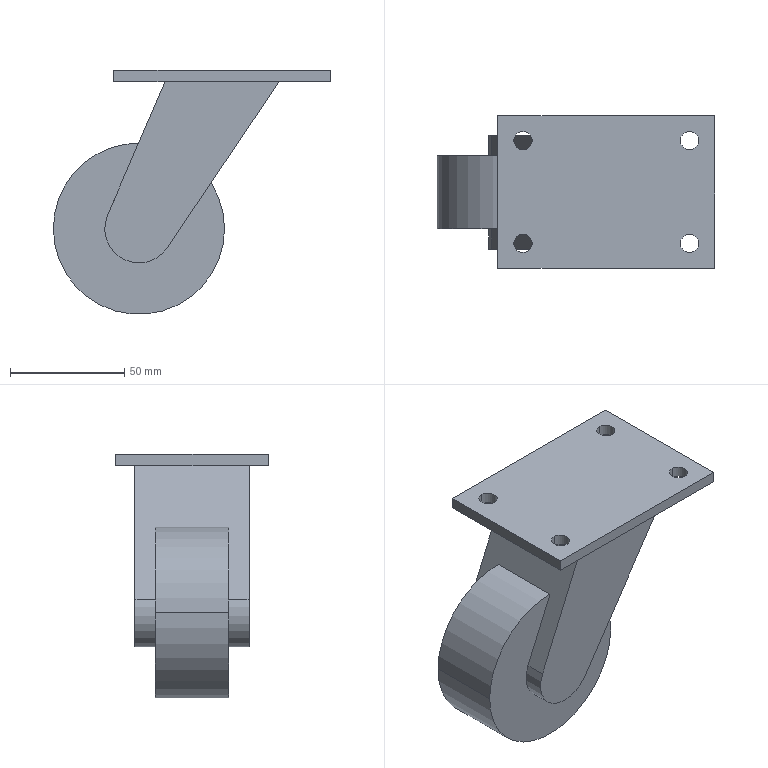Component | SolidWorks | Caster-3 | 1 solid | 25 faces | box 121.5 x 67 x 107 mm | volume 276484 mm3 | cylinder 13 | plane 12 | commonest cylinder face diameters 8 x8 75 x3 30 x2
build123d program:
from build123d import *

# Parameters (mm, degrees)
SKETCH1_R          = 37.5
EXTRUDE1_DEPTH     = 16
SKETCH3_W          = 95
SKETCH3_H          = 5
EXTRUDE2_DEPTH     = 33.5
EXTRUDE3_DEPTH     = 25
CUT_EXTRUDE1_REACH = 142.097
SKETCH5_R          = 4


with BuildPart() as part:
    # Sketch1 → Extrude1 (new, symmetric)
    with BuildSketch(Plane.XY):
        Circle(SKETCH1_R)
    extrude(amount=EXTRUDE1_DEPTH, both=True)



with BuildPart() as body_2:
    # Sketch3 → Extrude2 (new, symmetric)
    with BuildSketch(Plane.XY):
        with Locations((-36.5, 67)):
            Rectangle(SKETCH3_W, SKETCH3_H)
    extrude(amount=EXTRUDE2_DEPTH, both=True)


with BuildPart() as part_1:
    add(part.part)

    add(body_2.part)  # Extrude3 merges body 2
    # Sketch4 → Extrude3 (add, symmetric)
    with BuildSketch(Plane.XY):
        with BuildLine():
            Line((-61.5, 64.5), (-11.5, 64.5))
            Line((-11.5, 64.5), (13.772, 5.944))
            ThreePointArc((13.772, 5.944), (7.191, -13.164), (-12.443, -8.376))
            Line((-12.443, -8.376), (-61.5, 64.5))
        make_face()
    extrude(amount=EXTRUDE3_DEPTH, both=True)

    # Sketch5 → Cut-Extrude1 (cut, up to next)
    with BuildSketch(Plane(origin=(0, 69.5, 0), x_dir=(-1, 0, 0), z_dir=(0, 1, 0)), mode=Mode.PRIVATE) as cut_extrude1_sk1:
        with Locations(Location((0, -22.5, 0), (0, 0, 90))):
            Circle(SKETCH5_R)
    cut_extrude1_tool1 = extrude(cut_extrude1_sk1.sketch, amount=-CUT_EXTRUDE1_REACH, mode=Mode.PRIVATE) & part_1.part
    # Sketch5 → Cut-Extrude1 (cut, up to next)
    with BuildSketch(Plane(origin=(0, 69.5, 0), x_dir=(-1, 0, 0), z_dir=(0, 1, 0)), mode=Mode.PRIVATE) as cut_extrude1_sk2:
        with Locations(Location((0, 22.5, 0), (0, 0, 90))):
            Circle(SKETCH5_R)
    cut_extrude1_tool2 = extrude(cut_extrude1_sk2.sketch, amount=-CUT_EXTRUDE1_REACH, mode=Mode.PRIVATE) & part_1.part
    # Sketch5 → Cut-Extrude1 (cut, up to next)
    with BuildSketch(Plane(origin=(0, 69.5, 0), x_dir=(-1, 0, 0), z_dir=(0, 1, 0)), mode=Mode.PRIVATE) as cut_extrude1_sk3:
        with Locations(Location((73, 22.5, 0), (0, 0, 90))):
            Circle(SKETCH5_R)
    cut_extrude1_tool3 = extrude(cut_extrude1_sk3.sketch, amount=-CUT_EXTRUDE1_REACH, mode=Mode.PRIVATE) & part_1.part
    # Sketch5 → Cut-Extrude1 (cut, up to next)
    with BuildSketch(Plane(origin=(0, 69.5, 0), x_dir=(-1, 0, 0), z_dir=(0, 1, 0)), mode=Mode.PRIVATE) as cut_extrude1_sk4:
        with Locations(Location((73, -22.5, 0), (0, 0, 90))):
            Circle(SKETCH5_R)
    cut_extrude1_tool4 = extrude(cut_extrude1_sk4.sketch, amount=-CUT_EXTRUDE1_REACH, mode=Mode.PRIVATE) & part_1.part
    add(cut_extrude1_tool1.solids().sort_by_distance((0, 69.5, -22.5))[0], mode=Mode.SUBTRACT)
    add(cut_extrude1_tool2.solids().sort_by_distance((0, 69.5, 22.5))[0], mode=Mode.SUBTRACT)
    add(cut_extrude1_tool3.solids().sort_by_distance((-73, 69.5, 22.5))[0], mode=Mode.SUBTRACT)
    add(cut_extrude1_tool4.solids().sort_by_distance((-73, 69.5, -22.5))[0], mode=Mode.SUBTRACT)


solid = part_1.part

# Placed as in the assembly
solid = solid.moved(Location((-626.868, -171.075, 1106.75), (-90, 0, 180)))
STEP:
#1=CARTESIAN_POINT('',(-21.806,-7.464,46.112));
#2=VERTEX_POINT('',#1);
#3=CARTESIAN_POINT('',(-21.806,-7.779,46.112));
#4=VERTEX_POINT('',#3);
#5=CARTESIAN_POINT('',(-21.806,-7.621,46.112));
#6=DIRECTION('',(-0.,-0.,-1.));
#7=DIRECTION('',(0.,1.,0.));
#8=AXIS2_PLACEMENT_3D('',#5,#6,#7);
#9=CIRCLE('',#8,0.1575);
#10=EDGE_CURVE('',#2,#4,#9,.T.);
#11=ORIENTED_EDGE('',*,*,#10,.T.);
#12=CARTESIAN_POINT('',(-21.806,-7.779,46.309));
#13=VERTEX_POINT('',#12);
#14=CARTESIAN_POINT('',(-21.806,-7.779,42.096));
#15=DIRECTION('',(0.,0.,1.));
#16=VECTOR('',#15,39.37);
#17=LINE('',#14,#16);
#18=EDGE_CURVE('',#4,#13,#17,.T.);
#19=ORIENTED_EDGE('',*,*,#18,.T.);
#20=CARTESIAN_POINT('',(-21.806,-7.464,46.309));
#21=VERTEX_POINT('',#20);
#22=CARTESIAN_POINT('',(-21.806,-7.621,46.309));
#23=DIRECTION('',(0.,0.,1.));
#24=DIRECTION('',(0.,1.,0.));
#25=AXIS2_PLACEMENT_3D('',#22,#23,#24);
#26=CIRCLE('',#25,0.1575);
#27=EDGE_CURVE('',#13,#21,#26,.T.);
#28=ORIENTED_EDGE('',*,*,#27,.T.);
#29=CARTESIAN_POINT('',(-21.806,-7.464,42.096));
#30=DIRECTION('',(0.,0.,1.));
#31=VECTOR('',#30,39.37);
#32=LINE('',#29,#31);
#33=EDGE_CURVE('',#2,#21,#32,.T.);
#34=ORIENTED_EDGE('',*,*,#33,.F.);
#35=EDGE_LOOP('',(#11,#19,#28,#34));
#36=FACE_OUTER_BOUND('',#35,.T.);
#37=CARTESIAN_POINT('',(-21.806,-7.621,42.096));
#38=DIRECTION('',(0.,0.,1.));
#39=DIRECTION('',(0.,1.,0.));
#40=AXIS2_PLACEMENT_3D('',#37,#38,#39);
#41=CYLINDRICAL_SURFACE('',#40,0.1575);
#42=ADVANCED_FACE('',(#36),#41,.F.);
#43=CARTESIAN_POINT('',(-21.806,-5.692,46.112));
#44=VERTEX_POINT('',#43);
#45=CARTESIAN_POINT('',(-21.806,-6.007,46.112));
#46=VERTEX_POINT('',#45);
#47=CARTESIAN_POINT('',(-21.806,-5.849,46.112));
#48=DIRECTION('',(-0.,-0.,-1.));
#49=DIRECTION('',(0.,1.,0.));
#50=AXIS2_PLACEMENT_3D('',#47,#48,#49);
#51=CIRCLE('',#50,0.1575);
#52=EDGE_CURVE('',#44,#46,#51,.T.);
#53=ORIENTED_EDGE('',*,*,#52,.T.);
#54=CARTESIAN_POINT('',(-21.806,-6.007,46.309));
#55=VERTEX_POINT('',#54);
#56=CARTESIAN_POINT('',(-21.806,-6.007,42.096));
#57=DIRECTION('',(0.,0.,1.));
#58=VECTOR('',#57,39.37);
#59=LINE('',#56,#58);
#60=EDGE_CURVE('',#46,#55,#59,.T.);
#61=ORIENTED_EDGE('',*,*,#60,.T.);
#62=CARTESIAN_POINT('',(-21.806,-5.692,46.309));
#63=VERTEX_POINT('',#62);
#64=CARTESIAN_POINT('',(-21.806,-5.849,46.309));
#65=DIRECTION('',(0.,0.,1.));
#66=DIRECTION('',(0.,1.,0.));
#67=AXIS2_PLACEMENT_3D('',#64,#65,#66);
#68=CIRCLE('',#67,0.1575);
#69=EDGE_CURVE('',#55,#63,#68,.T.);
#70=ORIENTED_EDGE('',*,*,#69,.T.);
#71=CARTESIAN_POINT('',(-21.806,-5.692,42.096));
#72=DIRECTION('',(0.,0.,1.));
#73=VECTOR('',#72,39.37);
#74=LINE('',#71,#73);
#75=EDGE_CURVE('',#44,#63,#74,.T.);
#76=ORIENTED_EDGE('',*,*,#75,.F.);
#77=EDGE_LOOP('',(#53,#61,#70,#76));
#78=FACE_OUTER_BOUND('',#77,.T.);
#79=CARTESIAN_POINT('',(-21.806,-5.849,42.096));
#80=DIRECTION('',(0.,0.,1.));
#81=DIRECTION('',(0.,1.,0.));
#82=AXIS2_PLACEMENT_3D('',#79,#80,#81);
#83=CYLINDRICAL_SURFACE('',#82,0.1575);
#84=ADVANCED_FACE('',(#78),#83,.F.);
#85=CARTESIAN_POINT('',(-24.68,-5.692,46.112));
#86=VERTEX_POINT('',#85);
#87=CARTESIAN_POINT('',(-24.68,-6.007,46.112));
#88=VERTEX_POINT('',#87);
#89=CARTESIAN_POINT('',(-24.68,-5.849,46.112));
#90=DIRECTION('',(-0.,-0.,-1.));
#91=DIRECTION('',(0.,1.,0.));
#92=AXIS2_PLACEMENT_3D('',#89,#90,#91);
#93=CIRCLE('',#92,0.1575);
#94=EDGE_CURVE('',#86,#88,#93,.T.);
#95=ORIENTED_EDGE('',*,*,#94,.T.);
#96=CARTESIAN_POINT('',(-24.68,-6.007,46.309));
#97=VERTEX_POINT('',#96);
#98=CARTESIAN_POINT('',(-24.68,-6.007,42.096));
#99=DIRECTION('',(0.,0.,1.));
#100=VECTOR('',#99,39.37);
#101=LINE('',#98,#100);
#102=EDGE_CURVE('',#88,#97,#101,.T.);
#103=ORIENTED_EDGE('',*,*,#102,.T.);
#104=CARTESIAN_POINT('',(-24.68,-5.692,46.309));
#105=VERTEX_POINT('',#104);
#106=CARTESIAN_POINT('',(-24.68,-5.849,46.309));
#107=DIRECTION('',(0.,0.,1.));
#108=DIRECTION('',(0.,1.,0.));
#109=AXIS2_PLACEMENT_3D('',#106,#107,#108);
#110=CIRCLE('',#109,0.1575);
#111=EDGE_CURVE('',#97,#105,#110,.T.);
#112=ORIENTED_EDGE('',*,*,#111,.T.);
#113=CARTESIAN_POINT('',(-24.68,-5.692,42.096));
#114=DIRECTION('',(0.,0.,1.));
#115=VECTOR('',#114,39.37);
#116=LINE('',#113,#115);
#117=EDGE_CURVE('',#86,#105,#116,.T.);
#118=ORIENTED_EDGE('',*,*,#117,.F.);
#119=EDGE_LOOP('',(#95,#103,#112,#118));
#120=FACE_OUTER_BOUND('',#119,.T.);
#121=CARTESIAN_POINT('',(-24.68,-5.849,42.096));
#122=DIRECTION('',(0.,0.,1.));
#123=DIRECTION('',(0.,1.,0.));
#124=AXIS2_PLACEMENT_3D('',#121,#122,#123);
#125=CYLINDRICAL_SURFACE('',#124,0.1575);
#126=ADVANCED_FACE('',(#120),#125,.F.);
#127=CARTESIAN_POINT('',(-24.68,-7.464,46.112));
#128=VERTEX_POINT('',#127);
#129=CARTESIAN_POINT('',(-24.68,-7.779,46.112));
#130=VERTEX_POINT('',#129);
#131=CARTESIAN_POINT('',(-24.68,-7.621,46.112));
#132=DIRECTION('',(-0.,-0.,-1.));
#133=DIRECTION('',(0.,1.,0.));
#134=AXIS2_PLACEMENT_3D('',#131,#132,#133);
#135=CIRCLE('',#134,0.1575);
#136=EDGE_CURVE('',#128,#130,#135,.T.);
#137=ORIENTED_EDGE('',*,*,#136,.T.);
#138=CARTESIAN_POINT('',(-24.68,-7.779,46.309));
#139=VERTEX_POINT('',#138);
#140=CARTESIAN_POINT('',(-24.68,-7.779,42.096));
#141=DIRECTION('',(0.,0.,1.));
#142=VECTOR('',#141,39.37);
#143=LINE('',#140,#142);
#144=EDGE_CURVE('',#130,#139,#143,.T.);
#145=ORIENTED_EDGE('',*,*,#144,.T.);
#146=CARTESIAN_POINT('',(-24.68,-7.464,46.309));
#147=VERTEX_POINT('',#146);
#148=CARTESIAN_POINT('',(-24.68,-7.621,46.309));
#149=DIRECTION('',(0.,0.,1.));
#150=DIRECTION('',(0.,1.,0.));
#151=AXIS2_PLACEMENT_3D('',#148,#149,#150);
#152=CIRCLE('',#151,0.1575);
#153=EDGE_CURVE('',#139,#147,#152,.T.);
#154=ORIENTED_EDGE('',*,*,#153,.T.);
#155=CARTESIAN_POINT('',(-24.68,-7.464,42.096));
#156=DIRECTION('',(0.,0.,1.));
#157=VECTOR('',#156,39.37);
#158=LINE('',#155,#157);
#159=EDGE_CURVE('',#128,#147,#158,.T.);
#160=ORIENTED_EDGE('',*,*,#159,.F.);
#161=EDGE_LOOP('',(#137,#145,#154,#160));
#162=FACE_OUTER_BOUND('',#161,.T.);
#163=CARTESIAN_POINT('',(-24.68,-7.621,42.096));
#164=DIRECTION('',(0.,0.,1.));
#165=DIRECTION('',(0.,1.,0.));
#166=AXIS2_PLACEMENT_3D('',#163,#164,#165);
#167=CYLINDRICAL_SURFACE('',#166,0.1575);
#168=ADVANCED_FACE('',(#162),#167,.F.);
#169=CARTESIAN_POINT('',(-26.156,-6.105,43.573));
#170=VERTEX_POINT('',#169);
#171=CARTESIAN_POINT('',(-24.686,-6.105,45.049));
#172=VERTEX_POINT('',#171);
#173=CARTESIAN_POINT('',(-24.68,-6.105,43.573));
#174=DIRECTION('',(0.,1.,-0.));
#175=DIRECTION('',(-1.,0.,0.));
#176=AXIS2_PLACEMENT_3D('',#173,#174,#175);
#177=CIRCLE('',#176,1.476);
#178=EDGE_CURVE('',#170,#172,#177,.T.);
#179=ORIENTED_EDGE('',*,*,#178,.F.);
#180=CARTESIAN_POINT('',(-26.156,-7.365,43.573));
#181=VERTEX_POINT('',#180);
#182=CARTESIAN_POINT('',(-26.156,-6.105,43.573));
#183=DIRECTION('',(-0.,-1.,0.));
#184=VECTOR('',#183,39.37);
#185=LINE('',#182,#184);
#186=EDGE_CURVE('',#170,#181,#185,.T.);
#187=ORIENTED_EDGE('',*,*,#186,.T.);
#188=CARTESIAN_POINT('',(-24.686,-7.365,45.049));
#189=VERTEX_POINT('',#188);
#190=CARTESIAN_POINT('',(-24.68,-7.365,43.573));
#191=DIRECTION('',(0.,1.,-0.));
#192=DIRECTION('',(-1.,0.,0.));
#193=AXIS2_PLACEMENT_3D('',#190,#191,#192);
#194=CIRCLE('',#193,1.476);
#195=EDGE_CURVE('',#181,#189,#194,.T.);
#196=ORIENTED_EDGE('',*,*,#195,.T.);
#197=CARTESIAN_POINT('',(-24.686,-6.105,45.049));
#198=DIRECTION('',(0.,1.,-0.));
#199=VECTOR('',#198,39.37);
#200=LINE('',#197,#199);
#201=EDGE_CURVE('',#189,#172,#200,.T.);
#202=ORIENTED_EDGE('',*,*,#201,.T.);
#203=EDGE_LOOP('',(#179,#187,#196,#202));
#204=FACE_OUTER_BOUND('',#203,.T.);
#205=CARTESIAN_POINT('',(-24.68,-6.105,43.573));
#206=DIRECTION('',(-0.,-1.,0.));
#207=DIRECTION('',(1.,-0.,0.));
#208=AXIS2_PLACEMENT_3D('',#205,#206,#207);
#209=CYLINDRICAL_SURFACE('',#208,1.476);
#210=ADVANCED_FACE('',(#204),#209,.T.);
#211=ORIENTED_EDGE('',*,*,#186,.F.);
#212=CARTESIAN_POINT('',(-23.203,-6.105,43.573));
#213=VERTEX_POINT('',#212);
#214=CARTESIAN_POINT('',(-24.68,-6.105,43.573));
#215=DIRECTION('',(0.,1.,-0.));
#216=DIRECTION('',(-1.,0.,0.));
#217=AXIS2_PLACEMENT_3D('',#214,#215,#216);
#218=CIRCLE('',#217,1.476);
#219=EDGE_CURVE('',#213,#170,#218,.T.);
#220=ORIENTED_EDGE('',*,*,#219,.F.);
#221=CARTESIAN_POINT('',(-23.203,-7.365,43.573));
#222=VERTEX_POINT('',#221);
#223=CARTESIAN_POINT('',(-23.203,-6.105,43.573));
#224=DIRECTION('',(-0.,-1.,0.));
#225=VECTOR('',#224,39.37);
#226=LINE('',#223,#225);
#227=EDGE_CURVE('',#213,#222,#226,.T.);
#228=ORIENTED_EDGE('',*,*,#227,.T.);
#229=CARTESIAN_POINT('',(-24.68,-7.365,43.573));
#230=DIRECTION('',(0.,1.,-0.));
#231=DIRECTION('',(-1.,0.,0.));
#232=AXIS2_PLACEMENT_3D('',#229,#230,#231);
#233=CIRCLE('',#232,1.476);
#234=EDGE_CURVE('',#222,#181,#233,.T.);
#235=ORIENTED_EDGE('',*,*,#234,.T.);
#236=EDGE_LOOP('',(#211,#220,#228,#235));
#237=FACE_OUTER_BOUND('',#236,.T.);
#238=CARTESIAN_POINT('',(-24.68,-6.105,43.573));
#239=DIRECTION('',(-0.,-1.,0.));
#240=DIRECTION('',(1.,-0.,0.));
#241=AXIS2_PLACEMENT_3D('',#238,#239,#240);
#242=CYLINDRICAL_SURFACE('',#241,1.476);
#243=ADVANCED_FACE('',(#237),#242,.T.);
#244=CARTESIAN_POINT('',(-24.19,-7.365,43.243));
#245=VERTEX_POINT('',#244);
#246=CARTESIAN_POINT('',(-25.222,-7.365,43.807));
#247=VERTEX_POINT('',#246);
#248=CARTESIAN_POINT('',(-24.68,-7.365,43.573));
#249=DIRECTION('',(0.,1.,-0.));
#250=DIRECTION('',(-1.,0.,0.));
#251=AXIS2_PLACEMENT_3D('',#248,#249,#250);
#252=CIRCLE('',#251,0.5906);
#253=EDGE_CURVE('',#245,#247,#252,.T.);
#254=ORIENTED_EDGE('',*,*,#253,.F.);
#255=CARTESIAN_POINT('',(-24.19,-7.72,43.243));
#256=VERTEX_POINT('',#255);
#257=CARTESIAN_POINT('',(-24.19,-5.751,43.243));
#258=DIRECTION('',(-0.,-1.,0.));
#259=VECTOR('',#258,39.37);
#260=LINE('',#257,#259);
#261=EDGE_CURVE('',#245,#256,#260,.T.);
#262=ORIENTED_EDGE('',*,*,#261,.T.);
#263=CARTESIAN_POINT('',(-25.222,-7.72,43.807));
#264=VERTEX_POINT('',#263);
#265=CARTESIAN_POINT('',(-24.68,-7.72,43.573));
#266=DIRECTION('',(0.,1.,-0.));
#267=DIRECTION('',(-1.,0.,0.));
#268=AXIS2_PLACEMENT_3D('',#265,#266,#267);
#269=CIRCLE('',#268,0.5906);
#270=EDGE_CURVE('',#256,#264,#269,.T.);
#271=ORIENTED_EDGE('',*,*,#270,.T.);
#272=CARTESIAN_POINT('',(-25.222,-5.751,43.807));
#273=DIRECTION('',(-0.,-1.,0.));
#274=VECTOR('',#273,39.37);
#275=LINE('',#272,#274);
#276=EDGE_CURVE('',#247,#264,#275,.T.);
#277=ORIENTED_EDGE('',*,*,#276,.F.);
#278=EDGE_LOOP('',(#254,#262,#271,#277));
#279=FACE_OUTER_BOUND('',#278,.T.);
#280=CARTESIAN_POINT('',(-24.68,-5.751,43.573));
#281=DIRECTION('',(-0.,-1.,0.));
#282=DIRECTION('',(1.,-0.,0.));
#283=AXIS2_PLACEMENT_3D('',#280,#281,#282);
#284=CYLINDRICAL_SURFACE('',#283,0.5906);
#285=ADVANCED_FACE('',(#279),#284,.T.);
#286=CARTESIAN_POINT('',(-21.373,-8.054,46.309));
#287=VERTEX_POINT('',#286);
#288=CARTESIAN_POINT('',(-21.373,-8.054,46.112));
#289=VERTEX_POINT('',#288);
#290=CARTESIAN_POINT('',(-21.373,-8.054,46.309));
#291=DIRECTION('',(-0.,-0.,-1.));
#292=VECTOR('',#291,39.37);
#293=LINE('',#290,#292);
#294=EDGE_CURVE('',#287,#289,#293,.T.);
#295=ORIENTED_EDGE('',*,*,#294,.T.);
#296=CARTESIAN_POINT('',(-21.373,-5.416,46.112));
#297=VERTEX_POINT('',#296);
#298=CARTESIAN_POINT('',(-21.373,-5.416,46.112));
#299=DIRECTION('',(-0.,-1.,0.));
#300=VECTOR('',#299,39.37);
#301=LINE('',#298,#300);
#302=EDGE_CURVE('',#297,#289,#301,.T.);
#303=ORIENTED_EDGE('',*,*,#302,.F.);
#304=CARTESIAN_POINT('',(-21.373,-5.416,46.309));
#305=VERTEX_POINT('',#304);
#306=CARTESIAN_POINT('',(-21.373,-5.416,46.309));
#307=DIRECTION('',(-0.,-0.,-1.));
#308=VECTOR('',#307,39.37);
#309=LINE('',#306,#308);
#310=EDGE_CURVE('',#305,#297,#309,.T.);
#311=ORIENTED_EDGE('',*,*,#310,.F.);
#312=CARTESIAN_POINT('',(-21.373,-5.416,46.309));
#313=DIRECTION('',(-0.,-1.,0.));
#314=VECTOR('',#313,39.37);
#315=LINE('',#312,#314);
#316=EDGE_CURVE('',#305,#287,#315,.T.);
#317=ORIENTED_EDGE('',*,*,#316,.T.);
#318=EDGE_LOOP('',(#295,#303,#311,#317));
#319=FACE_OUTER_BOUND('',#318,.T.);
#320=CARTESIAN_POINT('',(-21.373,-5.416,46.309));
#321=DIRECTION('',(-1.,0.,0.));
#322=DIRECTION('',(-0.,-1.,0.));
#323=AXIS2_PLACEMENT_3D('',#320,#321,#322);
#324=PLANE('',#323);
#325=ADVANCED_FACE('',(#319),#324,.F.);
#326=ORIENTED_EDGE('',*,*,#10,.F.);
#327=CARTESIAN_POINT('',(-21.806,-7.621,46.112));
#328=DIRECTION('',(-0.,-0.,-1.));
#329=DIRECTION('',(0.,1.,0.));
#330=AXIS2_PLACEMENT_3D('',#327,#328,#329);
#331=CIRCLE('',#330,0.1575);
#332=EDGE_CURVE('',#4,#2,#331,.T.);
#333=ORIENTED_EDGE('',*,*,#332,.F.);
#334=EDGE_LOOP('',(#326,#333));
#335=FACE_BOUND('',#334,.T.);
#336=ORIENTED_EDGE('',*,*,#52,.F.);
#337=CARTESIAN_POINT('',(-21.806,-5.849,46.112));
#338=DIRECTION('',(-0.,-0.,-1.));
#339=DIRECTION('',(0.,1.,0.));
#340=AXIS2_PLACEMENT_3D('',#337,#338,#339);
#341=CIRCLE('',#340,0.1575);
#342=EDGE_CURVE('',#46,#44,#341,.T.);
#343=ORIENTED_EDGE('',*,*,#342,.F.);
#344=EDGE_LOOP('',(#336,#343));
#345=FACE_BOUND('',#344,.T.);
#346=ORIENTED_EDGE('',*,*,#94,.F.);
#347=CARTESIAN_POINT('',(-24.68,-5.849,46.112));
#348=DIRECTION('',(-0.,-0.,-1.));
#349=DIRECTION('',(0.,1.,0.));
#350=AXIS2_PLACEMENT_3D('',#347,#348,#349);
#351=CIRCLE('',#350,0.1575);
#352=EDGE_CURVE('',#88,#86,#351,.T.);
#353=ORIENTED_EDGE('',*,*,#352,.F.);
#354=EDGE_LOOP('',(#346,#353));
#355=FACE_BOUND('',#354,.T.);
#356=ORIENTED_EDGE('',*,*,#136,.F.);
#357=CARTESIAN_POINT('',(-24.68,-7.621,46.112));
#358=DIRECTION('',(-0.,-0.,-1.));
#359=DIRECTION('',(0.,1.,0.));
#360=AXIS2_PLACEMENT_3D('',#357,#358,#359);
#361=CIRCLE('',#360,0.1575);
#362=EDGE_CURVE('',#130,#128,#361,.T.);
#363=ORIENTED_EDGE('',*,*,#362,.F.);
#364=EDGE_LOOP('',(#356,#363));
#365=FACE_BOUND('',#364,.T.);
#366=CARTESIAN_POINT('',(-22.259,-5.751,46.112));
#367=VERTEX_POINT('',#366);
#368=CARTESIAN_POINT('',(-22.259,-7.72,46.112));
#369=VERTEX_POINT('',#368);
#370=CARTESIAN_POINT('',(-22.259,-5.751,46.112));
#371=DIRECTION('',(-0.,-1.,0.));
#372=VECTOR('',#371,39.37);
#373=LINE('',#370,#372);
#374=EDGE_CURVE('',#367,#369,#373,.T.);
#375=ORIENTED_EDGE('',*,*,#374,.F.);
#376=CARTESIAN_POINT('',(-24.227,-5.751,46.112));
#377=VERTEX_POINT('',#376);
#378=CARTESIAN_POINT('',(-22.259,-5.751,46.112));
#379=DIRECTION('',(1.,-0.,-0.));
#380=VECTOR('',#379,39.37);
#381=LINE('',#378,#380);
#382=EDGE_CURVE('',#377,#367,#381,.T.);
#383=ORIENTED_EDGE('',*,*,#382,.F.);
#384=CARTESIAN_POINT('',(-24.227,-7.72,46.112));
#385=VERTEX_POINT('',#384);
#386=CARTESIAN_POINT('',(-24.227,-5.751,46.112));
#387=DIRECTION('',(-0.,-1.,0.));
#388=VECTOR('',#387,39.37);
#389=LINE('',#386,#388);
#390=EDGE_CURVE('',#377,#385,#389,.T.);
#391=ORIENTED_EDGE('',*,*,#390,.T.);
#392=CARTESIAN_POINT('',(-22.259,-7.72,46.112));
#393=DIRECTION('',(1.,-0.,-0.));
#394=VECTOR('',#393,39.37);
#395=LINE('',#392,#394);
#396=EDGE_CURVE('',#385,#369,#395,.T.);
#397=ORIENTED_EDGE('',*,*,#396,.T.);
#398=EDGE_LOOP('',(#375,#383,#391,#397));
#399=FACE_BOUND('',#398,.T.);
#400=CARTESIAN_POINT('',(-25.113,-8.054,46.112));
#401=VERTEX_POINT('',#400);
#402=CARTESIAN_POINT('',(-21.373,-8.054,46.112));
#403=DIRECTION('',(-1.,0.,0.));
#404=VECTOR('',#403,39.37);
#405=LINE('',#402,#404);
#406=EDGE_CURVE('',#289,#401,#405,.T.);
#407=ORIENTED_EDGE('',*,*,#406,.T.);
#408=CARTESIAN_POINT('',(-25.113,-5.416,46.112));
#409=VERTEX_POINT('',#408);
#410=CARTESIAN_POINT('',(-25.113,-5.416,46.112));
#411=DIRECTION('',(-0.,-1.,0.));
#412=VECTOR('',#411,39.37);
#413=LINE('',#410,#412);
#414=EDGE_CURVE('',#409,#401,#413,.T.);
#415=ORIENTED_EDGE('',*,*,#414,.F.);
#416=CARTESIAN_POINT('',(-21.373,-5.416,46.112));
#417=DIRECTION('',(-1.,0.,0.));
#418=VECTOR('',#417,39.37);
#419=LINE('',#416,#418);
#420=EDGE_CURVE('',#297,#409,#419,.T.);
#421=ORIENTED_EDGE('',*,*,#420,.F.);
#422=ORIENTED_EDGE('',*,*,#302,.T.);
#423=EDGE_LOOP('',(#407,#415,#421,#422));
#424=FACE_OUTER_BOUND('',#423,.T.);
#425=CARTESIAN_POINT('',(-21.373,-5.416,46.112));
#426=DIRECTION('',(0.,0.,1.));
#427=DIRECTION('',(0.,1.,-0.));
#428=AXIS2_PLACEMENT_3D('',#425,#426,#427);
#429=PLANE('',#428);
#430=ADVANCED_FACE('',(#335,#345,#355,#365,#399,#424),#429,.F.);
#431=CARTESIAN_POINT('',(-25.113,-8.054,46.309));
#432=VERTEX_POINT('',#431);
#433=CARTESIAN_POINT('',(-25.113,-8.054,46.309));
#434=DIRECTION('',(0.,0.,1.));
#435=VECTOR('',#434,39.37);
#436=LINE('',#433,#435);
#437=EDGE_CURVE('',#401,#432,#436,.T.);
#438=ORIENTED_EDGE('',*,*,#437,.T.);
#439=CARTESIAN_POINT('',(-25.113,-5.416,46.309));
#440=VERTEX_POINT('',#439);
#441=CARTESIAN_POINT('',(-25.113,-5.416,46.309));
#442=DIRECTION('',(-0.,-1.,0.));
#443=VECTOR('',#442,39.37);
#444=LINE('',#441,#443);
#445=EDGE_CURVE('',#440,#432,#444,.T.);
#446=ORIENTED_EDGE('',*,*,#445,.F.);
#447=CARTESIAN_POINT('',(-25.113,-5.416,46.309));
#448=DIRECTION('',(0.,0.,1.));
#449=VECTOR('',#448,39.37);
#450=LINE('',#447,#449);
#451=EDGE_CURVE('',#409,#440,#450,.T.);
#452=ORIENTED_EDGE('',*,*,#451,.F.);
#453=ORIENTED_EDGE('',*,*,#414,.T.);
#454=EDGE_LOOP('',(#438,#446,#452,#453));
#455=FACE_OUTER_BOUND('',#454,.T.);
#456=CARTESIAN_POINT('',(-25.113,-5.416,46.309));
#457=DIRECTION('',(1.,-0.,-0.));
#458=DIRECTION('',(0.,1.,-0.));
#459=AXIS2_PLACEMENT_3D('',#456,#457,#458);
#460=PLANE('',#459);
#461=ADVANCED_FACE('',(#455),#460,.F.);
#462=CARTESIAN_POINT('',(-21.806,-7.621,46.309));
#463=DIRECTION('',(0.,0.,1.));
#464=DIRECTION('',(0.,1.,0.));
#465=AXIS2_PLACEMENT_3D('',#462,#463,#464);
#466=CIRCLE('',#465,0.1575);
#467=EDGE_CURVE('',#21,#13,#466,.T.);
#468=ORIENTED_EDGE('',*,*,#467,.F.);
#469=ORIENTED_EDGE('',*,*,#27,.F.);
#470=EDGE_LOOP('',(#468,#469));
#471=FACE_BOUND('',#470,.T.);
#472=CARTESIAN_POINT('',(-21.806,-5.849,46.309));
#473=DIRECTION('',(0.,0.,1.));
#474=DIRECTION('',(0.,1.,0.));
#475=AXIS2_PLACEMENT_3D('',#472,#473,#474);
#476=CIRCLE('',#475,0.1575);
#477=EDGE_CURVE('',#63,#55,#476,.T.);
#478=ORIENTED_EDGE('',*,*,#477,.F.);
#479=ORIENTED_EDGE('',*,*,#69,.F.);
#480=EDGE_LOOP('',(#478,#479));
#481=FACE_BOUND('',#480,.T.);
#482=CARTESIAN_POINT('',(-24.68,-5.849,46.309));
#483=DIRECTION('',(0.,0.,1.));
#484=DIRECTION('',(0.,1.,0.));
#485=AXIS2_PLACEMENT_3D('',#482,#483,#484);
#486=CIRCLE('',#485,0.1575);
#487=EDGE_CURVE('',#105,#97,#486,.T.);
#488=ORIENTED_EDGE('',*,*,#487,.F.);
#489=ORIENTED_EDGE('',*,*,#111,.F.);
#490=EDGE_LOOP('',(#488,#489));
#491=FACE_BOUND('',#490,.T.);
#492=CARTESIAN_POINT('',(-24.68,-7.621,46.309));
#493=DIRECTION('',(0.,0.,1.));
#494=DIRECTION('',(0.,1.,0.));
#495=AXIS2_PLACEMENT_3D('',#492,#493,#494);
#496=CIRCLE('',#495,0.1575);
#497=EDGE_CURVE('',#147,#139,#496,.T.);
#498=ORIENTED_EDGE('',*,*,#497,.F.);
#499=ORIENTED_EDGE('',*,*,#153,.F.);
#500=EDGE_LOOP('',(#498,#499));
#501=FACE_BOUND('',#500,.T.);
#502=CARTESIAN_POINT('',(-21.373,-8.054,46.309));
#503=DIRECTION('',(1.,-0.,-0.));
#504=VECTOR('',#503,39.37);
#505=LINE('',#502,#504);
#506=EDGE_CURVE('',#432,#287,#505,.T.);
#507=ORIENTED_EDGE('',*,*,#506,.T.);
#508=ORIENTED_EDGE('',*,*,#316,.F.);
#509=CARTESIAN_POINT('',(-21.373,-5.416,46.309));
#510=DIRECTION('',(1.,-0.,-0.));
#511=VECTOR('',#510,39.37);
#512=LINE('',#509,#511);
#513=EDGE_CURVE('',#440,#305,#512,.T.);
#514=ORIENTED_EDGE('',*,*,#513,.F.);
#515=ORIENTED_EDGE('',*,*,#445,.T.);
#516=EDGE_LOOP('',(#507,#508,#514,#515));
#517=FACE_OUTER_BOUND('',#516,.T.);
#518=CARTESIAN_POINT('',(-21.373,-5.416,46.309));
#519=DIRECTION('',(-0.,-0.,-1.));
#520=DIRECTION('',(-0.,-1.,0.));
#521=AXIS2_PLACEMENT_3D('',#518,#519,#520);
#522=PLANE('',#521);
#523=ADVANCED_FACE('',(#471,#481,#491,#501,#517),#522,.F.);
#524=ORIENTED_EDGE('',*,*,#310,.T.);
#525=ORIENTED_EDGE('',*,*,#420,.T.);
#526=ORIENTED_EDGE('',*,*,#451,.T.);
#527=ORIENTED_EDGE('',*,*,#513,.T.);
#528=EDGE_LOOP('',(#524,#525,#526,#527));
#529=FACE_OUTER_BOUND('',#528,.T.);
#530=CARTESIAN_POINT('',(-21.373,-5.416,46.112));
#531=DIRECTION('',(0.,1.,-0.));
#532=DIRECTION('',(-1.,0.,0.));
#533=AXIS2_PLACEMENT_3D('',#530,#531,#532);
#534=PLANE('',#533);
#535=ADVANCED_FACE('',(#529),#534,.T.);
#536=ORIENTED_EDGE('',*,*,#294,.F.);
#537=ORIENTED_EDGE('',*,*,#506,.F.);
#538=ORIENTED_EDGE('',*,*,#437,.F.);
#539=ORIENTED_EDGE('',*,*,#406,.F.);
#540=EDGE_LOOP('',(#536,#537,#538,#539));
#541=FACE_OUTER_BOUND('',#540,.T.);
#542=CARTESIAN_POINT('',(-21.373,-8.054,46.112));
#543=DIRECTION('',(0.,1.,-0.));
#544=DIRECTION('',(-1.,0.,0.));
#545=AXIS2_PLACEMENT_3D('',#542,#543,#544);
#546=PLANE('',#545);
#547=ADVANCED_FACE('',(#541),#546,.F.);
#548=CARTESIAN_POINT('',(-23.434,-6.105,44.366));
#549=VERTEX_POINT('',#548);
#550=CARTESIAN_POINT('',(-23.434,-7.365,44.366));
#551=VERTEX_POINT('',#550);
#552=CARTESIAN_POINT('',(-23.434,-6.105,44.366));
#553=DIRECTION('',(-0.,-1.,0.));
#554=VECTOR('',#553,39.37);
#555=LINE('',#552,#554);
#556=EDGE_CURVE('',#549,#551,#555,.T.);
#557=ORIENTED_EDGE('',*,*,#556,.F.);
#558=CARTESIAN_POINT('',(-24.19,-6.105,43.243));
#559=VERTEX_POINT('',#558);
#560=CARTESIAN_POINT('',(-22.259,-6.105,46.112));
#561=DIRECTION('',(-0.5584,0.,-0.8296));
#562=VECTOR('',#561,39.37);
#563=LINE('',#560,#562);
#564=EDGE_CURVE('',#549,#559,#563,.T.);
#565=ORIENTED_EDGE('',*,*,#564,.T.);
#566=CARTESIAN_POINT('',(-24.19,-5.751,43.243));
#567=VERTEX_POINT('',#566);
#568=CARTESIAN_POINT('',(-24.19,-5.751,43.243));
#569=DIRECTION('',(-0.,-1.,0.));
#570=VECTOR('',#569,39.37);
#571=LINE('',#568,#570);
#572=EDGE_CURVE('',#567,#559,#571,.T.);
#573=ORIENTED_EDGE('',*,*,#572,.F.);
#574=CARTESIAN_POINT('',(-22.259,-5.751,46.112));
#575=DIRECTION('',(-0.5584,0.,-0.8296));
#576=VECTOR('',#575,39.37);
#577=LINE('',#574,#576);
#578=EDGE_CURVE('',#367,#567,#577,.T.);
#579=ORIENTED_EDGE('',*,*,#578,.F.);
#580=ORIENTED_EDGE('',*,*,#374,.T.);
#581=CARTESIAN_POINT('',(-22.259,-7.72,46.112));
#582=DIRECTION('',(-0.5584,0.,-0.8296));
#583=VECTOR('',#582,39.37);
#584=LINE('',#581,#583);
#585=EDGE_CURVE('',#369,#256,#584,.T.);
#586=ORIENTED_EDGE('',*,*,#585,.T.);
#587=ORIENTED_EDGE('',*,*,#261,.F.);
#588=CARTESIAN_POINT('',(-22.259,-7.365,46.112));
#589=DIRECTION('',(-0.5584,0.,-0.8296));
#590=VECTOR('',#589,39.37);
#591=LINE('',#588,#590);
#592=EDGE_CURVE('',#551,#245,#591,.T.);
#593=ORIENTED_EDGE('',*,*,#592,.F.);
#594=EDGE_LOOP('',(#557,#565,#573,#579,#580,#586,#587,#593));
#595=FACE_OUTER_BOUND('',#594,.T.);
#596=CARTESIAN_POINT('',(-22.259,-5.751,46.112));
#597=DIRECTION('',(-0.8296,0.,0.5584));
#598=DIRECTION('',(0.5584,-0.,0.8296));
#599=AXIS2_PLACEMENT_3D('',#596,#597,#598);
#600=PLANE('',#599);
#601=ADVANCED_FACE('',(#595),#600,.F.);
#602=ORIENTED_EDGE('',*,*,#572,.T.);
#603=CARTESIAN_POINT('',(-25.222,-6.105,43.807));
#604=VERTEX_POINT('',#603);
#605=CARTESIAN_POINT('',(-24.68,-6.105,43.573));
#606=DIRECTION('',(0.,1.,-0.));
#607=DIRECTION('',(-1.,0.,0.));
#608=AXIS2_PLACEMENT_3D('',#605,#606,#607);
#609=CIRCLE('',#608,0.5906);
#610=EDGE_CURVE('',#559,#604,#609,.T.);
#611=ORIENTED_EDGE('',*,*,#610,.T.);
#612=CARTESIAN_POINT('',(-25.222,-5.751,43.807));
#613=VERTEX_POINT('',#612);
#614=CARTESIAN_POINT('',(-25.222,-5.751,43.807));
#615=DIRECTION('',(-0.,-1.,0.));
#616=VECTOR('',#615,39.37);
#617=LINE('',#614,#616);
#618=EDGE_CURVE('',#613,#604,#617,.T.);
#619=ORIENTED_EDGE('',*,*,#618,.F.);
#620=CARTESIAN_POINT('',(-24.68,-5.751,43.573));
#621=DIRECTION('',(0.,1.,-0.));
#622=DIRECTION('',(-1.,0.,0.));
#623=AXIS2_PLACEMENT_3D('',#620,#621,#622);
#624=CIRCLE('',#623,0.5906);
#625=EDGE_CURVE('',#567,#613,#624,.T.);
#626=ORIENTED_EDGE('',*,*,#625,.F.);
#627=EDGE_LOOP('',(#602,#611,#619,#626));
#628=FACE_OUTER_BOUND('',#627,.T.);
#629=CARTESIAN_POINT('',(-24.68,-5.751,43.573));
#630=DIRECTION('',(-0.,-1.,0.));
#631=DIRECTION('',(1.,-0.,0.));
#632=AXIS2_PLACEMENT_3D('',#629,#630,#631);
#633=CYLINDRICAL_SURFACE('',#632,0.5906);
#634=ADVANCED_FACE('',(#628),#633,.T.);
#635=ORIENTED_EDGE('',*,*,#618,.T.);
#636=CARTESIAN_POINT('',(-24.227,-6.105,46.112));
#637=DIRECTION('',(0.3963,-0.,0.9181));
#638=VECTOR('',#637,39.37);
#639=LINE('',#636,#638);
#640=EDGE_CURVE('',#604,#172,#639,.T.);
#641=ORIENTED_EDGE('',*,*,#640,.T.);
#642=ORIENTED_EDGE('',*,*,#201,.F.);
#643=CARTESIAN_POINT('',(-24.227,-7.365,46.112));
#644=DIRECTION('',(0.3963,-0.,0.9181));
#645=VECTOR('',#644,39.37);
#646=LINE('',#643,#645);
#647=EDGE_CURVE('',#247,#189,#646,.T.);
#648=ORIENTED_EDGE('',*,*,#647,.F.);
#649=ORIENTED_EDGE('',*,*,#276,.T.);
#650=CARTESIAN_POINT('',(-24.227,-7.72,46.112));
#651=DIRECTION('',(0.3963,-0.,0.9181));
#652=VECTOR('',#651,39.37);
#653=LINE('',#650,#652);
#654=EDGE_CURVE('',#264,#385,#653,.T.);
#655=ORIENTED_EDGE('',*,*,#654,.T.);
#656=ORIENTED_EDGE('',*,*,#390,.F.);
#657=CARTESIAN_POINT('',(-24.227,-5.751,46.112));
#658=DIRECTION('',(0.3963,-0.,0.9181));
#659=VECTOR('',#658,39.37);
#660=LINE('',#657,#659);
#661=EDGE_CURVE('',#613,#377,#660,.T.);
#662=ORIENTED_EDGE('',*,*,#661,.F.);
#663=EDGE_LOOP('',(#635,#641,#642,#648,#649,#655,#656,#662));
#664=FACE_OUTER_BOUND('',#663,.T.);
#665=CARTESIAN_POINT('',(-24.227,-5.751,46.112));
#666=DIRECTION('',(0.9181,-0.,-0.3963));
#667=DIRECTION('',(-0.3963,0.,-0.9181));
#668=AXIS2_PLACEMENT_3D('',#665,#666,#667);
#669=PLANE('',#668);
#670=ADVANCED_FACE('',(#664),#669,.F.);
#671=ORIENTED_EDGE('',*,*,#578,.T.);
#672=ORIENTED_EDGE('',*,*,#625,.T.);
#673=ORIENTED_EDGE('',*,*,#661,.T.);
#674=ORIENTED_EDGE('',*,*,#382,.T.);
#675=EDGE_LOOP('',(#671,#672,#673,#674));
#676=FACE_OUTER_BOUND('',#675,.T.);
#677=CARTESIAN_POINT('',(-24.68,-5.751,43.573));
#678=DIRECTION('',(0.,1.,-0.));
#679=DIRECTION('',(-1.,0.,0.));
#680=AXIS2_PLACEMENT_3D('',#677,#678,#679);
#681=PLANE('',#680);
#682=ADVANCED_FACE('',(#676),#681,.T.);
#683=ORIENTED_EDGE('',*,*,#585,.F.);
#684=ORIENTED_EDGE('',*,*,#396,.F.);
#685=ORIENTED_EDGE('',*,*,#654,.F.);
#686=ORIENTED_EDGE('',*,*,#270,.F.);
#687=EDGE_LOOP('',(#683,#684,#685,#686));
#688=FACE_OUTER_BOUND('',#687,.T.);
#689=CARTESIAN_POINT('',(-24.68,-7.72,43.573));
#690=DIRECTION('',(0.,1.,-0.));
#691=DIRECTION('',(-1.,0.,0.));
#692=AXIS2_PLACEMENT_3D('',#689,#690,#691);
#693=PLANE('',#692);
#694=ADVANCED_FACE('',(#688),#693,.F.);
#695=ORIENTED_EDGE('',*,*,#227,.F.);
#696=CARTESIAN_POINT('',(-24.68,-6.105,43.573));
#697=DIRECTION('',(0.,1.,-0.));
#698=DIRECTION('',(-1.,0.,0.));
#699=AXIS2_PLACEMENT_3D('',#696,#697,#698);
#700=CIRCLE('',#699,1.476);
#701=EDGE_CURVE('',#549,#213,#700,.T.);
#702=ORIENTED_EDGE('',*,*,#701,.F.);
#703=ORIENTED_EDGE('',*,*,#556,.T.);
#704=CARTESIAN_POINT('',(-24.68,-7.365,43.573));
#705=DIRECTION('',(0.,1.,-0.));
#706=DIRECTION('',(-1.,0.,0.));
#707=AXIS2_PLACEMENT_3D('',#704,#705,#706);
#708=CIRCLE('',#707,1.476);
#709=EDGE_CURVE('',#551,#222,#708,.T.);
#710=ORIENTED_EDGE('',*,*,#709,.T.);
#711=EDGE_LOOP('',(#695,#702,#703,#710));
#712=FACE_OUTER_BOUND('',#711,.T.);
#713=CARTESIAN_POINT('',(-24.68,-6.105,43.573));
#714=DIRECTION('',(-0.,-1.,0.));
#715=DIRECTION('',(1.,-0.,0.));
#716=AXIS2_PLACEMENT_3D('',#713,#714,#715);
#717=CYLINDRICAL_SURFACE('',#716,1.476);
#718=ADVANCED_FACE('',(#712),#717,.T.);
#719=ORIENTED_EDGE('',*,*,#564,.F.);
#720=ORIENTED_EDGE('',*,*,#701,.T.);
#721=ORIENTED_EDGE('',*,*,#219,.T.);
#722=ORIENTED_EDGE('',*,*,#178,.T.);
#723=ORIENTED_EDGE('',*,*,#640,.F.);
#724=ORIENTED_EDGE('',*,*,#610,.F.);
#725=EDGE_LOOP('',(#719,#720,#721,#722,#723,#724));
#726=FACE_OUTER_BOUND('',#725,.T.);
#727=CARTESIAN_POINT('',(-24.68,-6.105,43.573));
#728=DIRECTION('',(0.,1.,-0.));
#729=DIRECTION('',(-1.,0.,0.));
#730=AXIS2_PLACEMENT_3D('',#727,#728,#729);
#731=PLANE('',#730);
#732=ADVANCED_FACE('',(#726),#731,.T.);
#733=ORIENTED_EDGE('',*,*,#709,.F.);
#734=ORIENTED_EDGE('',*,*,#592,.T.);
#735=ORIENTED_EDGE('',*,*,#253,.T.);
#736=ORIENTED_EDGE('',*,*,#647,.T.);
#737=ORIENTED_EDGE('',*,*,#195,.F.);
#738=ORIENTED_EDGE('',*,*,#234,.F.);
#739=EDGE_LOOP('',(#733,#734,#735,#736,#737,#738));
#740=FACE_OUTER_BOUND('',#739,.T.);
#741=CARTESIAN_POINT('',(-24.68,-7.365,43.573));
#742=DIRECTION('',(0.,1.,-0.));
#743=DIRECTION('',(-1.,0.,0.));
#744=AXIS2_PLACEMENT_3D('',#741,#742,#743);
#745=PLANE('',#744);
#746=ADVANCED_FACE('',(#740),#745,.F.);
#747=ORIENTED_EDGE('',*,*,#144,.F.);
#748=ORIENTED_EDGE('',*,*,#362,.T.);
#749=ORIENTED_EDGE('',*,*,#159,.T.);
#750=ORIENTED_EDGE('',*,*,#497,.T.);
#751=EDGE_LOOP('',(#747,#748,#749,#750));
#752=FACE_OUTER_BOUND('',#751,.T.);
#753=CARTESIAN_POINT('',(-24.68,-7.621,42.096));
#754=DIRECTION('',(0.,0.,1.));
#755=DIRECTION('',(0.,1.,0.));
#756=AXIS2_PLACEMENT_3D('',#753,#754,#755);
#757=CYLINDRICAL_SURFACE('',#756,0.1575);
#758=ADVANCED_FACE('',(#752),#757,.F.);
#759=ORIENTED_EDGE('',*,*,#102,.F.);
#760=ORIENTED_EDGE('',*,*,#352,.T.);
#761=ORIENTED_EDGE('',*,*,#117,.T.);
#762=ORIENTED_EDGE('',*,*,#487,.T.);
#763=EDGE_LOOP('',(#759,#760,#761,#762));
#764=FACE_OUTER_BOUND('',#763,.T.);
#765=CARTESIAN_POINT('',(-24.68,-5.849,42.096));
#766=DIRECTION('',(0.,0.,1.));
#767=DIRECTION('',(0.,1.,0.));
#768=AXIS2_PLACEMENT_3D('',#765,#766,#767);
#769=CYLINDRICAL_SURFACE('',#768,0.1575);
#770=ADVANCED_FACE('',(#764),#769,.F.);
#771=ORIENTED_EDGE('',*,*,#60,.F.);
#772=ORIENTED_EDGE('',*,*,#342,.T.);
#773=ORIENTED_EDGE('',*,*,#75,.T.);
#774=ORIENTED_EDGE('',*,*,#477,.T.);
#775=EDGE_LOOP('',(#771,#772,#773,#774));
#776=FACE_OUTER_BOUND('',#775,.T.);
#777=CARTESIAN_POINT('',(-21.806,-5.849,42.096));
#778=DIRECTION('',(0.,0.,1.));
#779=DIRECTION('',(0.,1.,0.));
#780=AXIS2_PLACEMENT_3D('',#777,#778,#779);
#781=CYLINDRICAL_SURFACE('',#780,0.1575);
#782=ADVANCED_FACE('',(#776),#781,.F.);
#783=ORIENTED_EDGE('',*,*,#18,.F.);
#784=ORIENTED_EDGE('',*,*,#332,.T.);
#785=ORIENTED_EDGE('',*,*,#33,.T.);
#786=ORIENTED_EDGE('',*,*,#467,.T.);
#787=EDGE_LOOP('',(#783,#784,#785,#786));
#788=FACE_OUTER_BOUND('',#787,.T.);
#789=CARTESIAN_POINT('',(-21.806,-7.621,42.096));
#790=DIRECTION('',(0.,0.,1.));
#791=DIRECTION('',(0.,1.,0.));
#792=AXIS2_PLACEMENT_3D('',#789,#790,#791);
#793=CYLINDRICAL_SURFACE('',#792,0.1575);
#794=ADVANCED_FACE('',(#788),#793,.F.);
#795=CLOSED_SHELL('',(#42,#84,#126,#168,#210,#243,#285,#325,#430,#461,#523,#535,#547,#601,#634,#670,#682,#694,#718,#732,#746,#758,#770,#782,#794));
#796=MANIFOLD_SOLID_BREP('',#795);
#797=CARTESIAN_POINT('',(0.,0.,0.));
#798=DIRECTION('',(0.,0.,1.));
#799=DIRECTION('',(1.,0.,0.));
#800=AXIS2_PLACEMENT_3D('',#797,#798,#799);
#801=(LENGTH_UNIT()NAMED_UNIT(*)SI_UNIT($,.METRE.));
#802=LENGTH_MEASURE_WITH_UNIT(LENGTH_MEASURE(0.0254),#801);
#803=DIMENSIONAL_EXPONENTS(1.,0.,0.,0.,0.,0.,0.);
#804=(CONVERSION_BASED_UNIT('',#802)LENGTH_UNIT()NAMED_UNIT(#803));
#805=UNCERTAINTY_MEASURE_WITH_UNIT(LENGTH_MEASURE(0.00001),#804,'','');
#806=(NAMED_UNIT(*)PLANE_ANGLE_UNIT()SI_UNIT($,.RADIAN.));
#807=(NAMED_UNIT(*)SI_UNIT($,.STERADIAN.)SOLID_ANGLE_UNIT());
#808=(GEOMETRIC_REPRESENTATION_CONTEXT(3)GLOBAL_UNCERTAINTY_ASSIGNED_CONTEXT((#805))GLOBAL_UNIT_ASSIGNED_CONTEXT((#804,#806,#807))REPRESENTATION_CONTEXT('',''));
#809=ADVANCED_BREP_SHAPE_REPRESENTATION('',(#796,#800),#808);
#810=COLOUR_RGB('',0.7922,0.8196,0.9333);
#811=FILL_AREA_STYLE_COLOUR('',#810);
#812=FILL_AREA_STYLE('',(#811));
#813=SURFACE_STYLE_FILL_AREA(#812);
#814=SURFACE_SIDE_STYLE('',(#813));
#815=SURFACE_STYLE_USAGE(.BOTH.,#814);
#816=PRESENTATION_STYLE_ASSIGNMENT((#815));
#817=STYLED_ITEM('',(#816),#796);
#818=(LENGTH_UNIT()NAMED_UNIT(*)SI_UNIT($,.METRE.));
#819=LENGTH_MEASURE_WITH_UNIT(LENGTH_MEASURE(0.0254),#818);
#820=DIMENSIONAL_EXPONENTS(1.,0.,0.,0.,0.,0.,0.);
#821=(CONVERSION_BASED_UNIT('',#819)LENGTH_UNIT()NAMED_UNIT(#820));
#822=UNCERTAINTY_MEASURE_WITH_UNIT(LENGTH_MEASURE(0.00001),#821,'','');
#823=(NAMED_UNIT(*)PLANE_ANGLE_UNIT()SI_UNIT($,.RADIAN.));
#824=(NAMED_UNIT(*)SI_UNIT($,.STERADIAN.)SOLID_ANGLE_UNIT());
#825=(GEOMETRIC_REPRESENTATION_CONTEXT(3)GLOBAL_UNCERTAINTY_ASSIGNED_CONTEXT((#822))GLOBAL_UNIT_ASSIGNED_CONTEXT((#821,#823,#824))REPRESENTATION_CONTEXT('',''));
#826=MECHANICAL_DESIGN_GEOMETRIC_PRESENTATION_REPRESENTATION('',(#817),#825);
#827=PRESENTATION_LAYER_ASSIGNMENT('','',(#817));